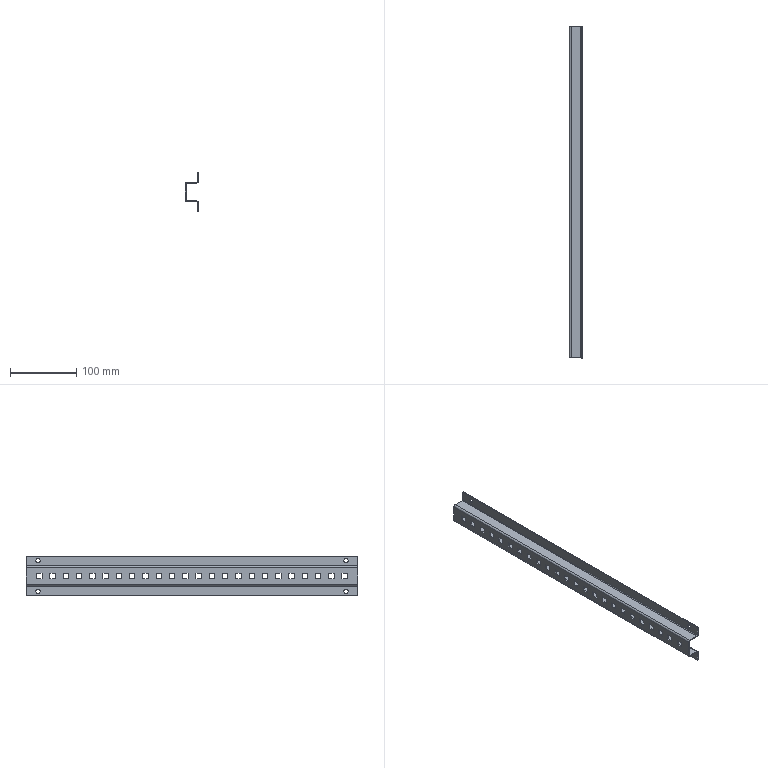Component | SolidWorks | GuidePlate-4 | 1 solid | 142 faces | volume 67877 mm3 | plane 126 | cylinder 16 | commonest cylinder face diameters 6.5 x8 2 x4 5 x4